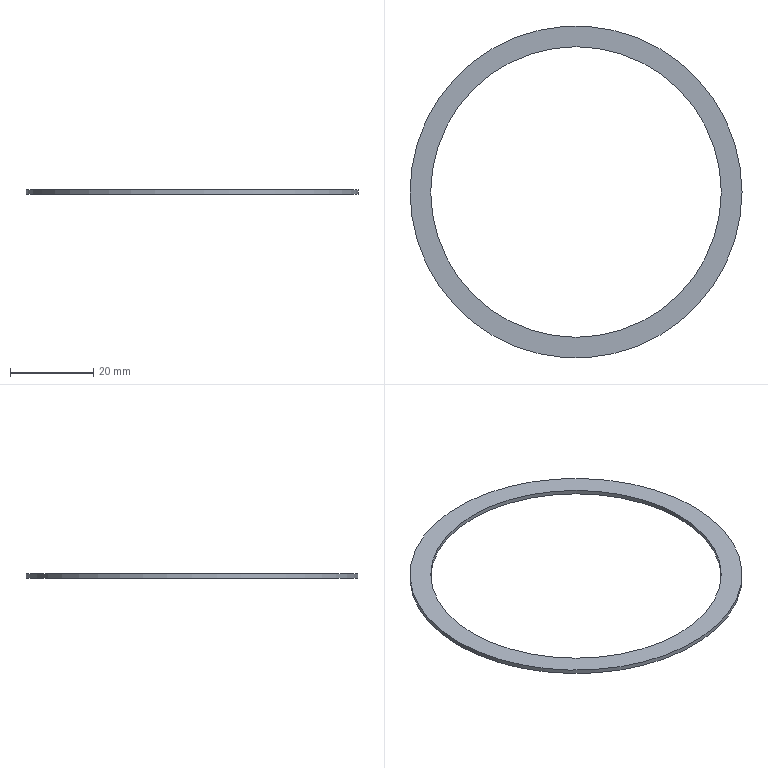Component | NX | BONNET_GASKET | 1 solid | 4 faces | box 80 x 80 x 1 mm | volume 1178 mm3 | plane 2 | cylinder 2 | commonest cylinder face diameters 80 x1 70 x1
STEP:
#1=CARTESIAN_POINT('',(0.,0.,0.));
#2=DIRECTION('',(0.,0.,1.));
#3=DIRECTION('',(1.,0.,0.));
#4=AXIS2_PLACEMENT_3D('',#1,#2,#3);
#5=CARTESIAN_POINT('',(35.,0.,-3.));
#6=VERTEX_POINT('',#5);
#7=CARTESIAN_POINT('',(0.,0.,-3.));
#8=DIRECTION('',(0.,0.,-1.));
#9=DIRECTION('',(1.,0.,0.));
#10=AXIS2_PLACEMENT_3D('',#7,#8,#9);
#11=CIRCLE('',#10,35.);
#12=CARTESIAN_POINT('',(0.,0.,-3.));
#13=DIRECTION('',(0.,0.,1.));
#14=DIRECTION('',(1.,0.,0.));
#15=AXIS2_PLACEMENT_3D('',#12,#13,#14);
#16=PLANE('',#15);
#17=CARTESIAN_POINT('',(35.,0.));
#18=CARTESIAN_POINT('',(35.,-60.622));
#19=CARTESIAN_POINT('',(-17.5,-30.311));
#20=CARTESIAN_POINT('',(-70.,-0.));
#21=CARTESIAN_POINT('',(-17.5,30.311));
#22=CARTESIAN_POINT('',(35.,60.622));
#23=CARTESIAN_POINT('',(35.,0.));
#24=(BOUNDED_CURVE()B_SPLINE_CURVE(2,(#17,#18,#19,#20,#21,#22,#23),.UNSPECIFIED.,.T.,.F.)B_SPLINE_CURVE_WITH_KNOTS((1,2,2,2,2,1),(-2.094,0.,2.094,4.189,6.283,8.378),.UNSPECIFIED.)CURVE()GEOMETRIC_REPRESENTATION_ITEM()RATIONAL_B_SPLINE_CURVE((1.,0.5,1.,0.5,1.,0.5,1.))REPRESENTATION_ITEM(''));
#25=(GEOMETRIC_REPRESENTATION_CONTEXT(2)PARAMETRIC_REPRESENTATION_CONTEXT()REPRESENTATION_CONTEXT('',''));
#26=DEFINITIONAL_REPRESENTATION('',(#24),#25);
#27=PCURVE('',#16,#26);
#28=CARTESIAN_POINT('',(0.,0.,-3.));
#29=DIRECTION('',(0.,0.,-1.));
#30=DIRECTION('',(1.,0.,0.));
#31=AXIS2_PLACEMENT_3D('',#28,#29,#30);
#32=CYLINDRICAL_SURFACE('',#31,35.);
#33=CARTESIAN_POINT('',(0.,0.));
#34=DIRECTION('',(1.,0.));
#35=VECTOR('',#34,1.);
#36=LINE('',#33,#35);
#37=(GEOMETRIC_REPRESENTATION_CONTEXT(2)PARAMETRIC_REPRESENTATION_CONTEXT()REPRESENTATION_CONTEXT('',''));
#38=DEFINITIONAL_REPRESENTATION('',(#36),#37);
#39=PCURVE('',#32,#38);
#40=SURFACE_CURVE('',#11,(#27,#39),.PCURVE_S1.);
#41=EDGE_CURVE('',#6,#6,#40,.T.);
#42=ORIENTED_EDGE('',*,*,#41,.T.);
#43=EDGE_LOOP('',(#42));
#44=FACE_BOUND('',#43,.T.);
#45=CARTESIAN_POINT('',(40.,0.,-3.));
#46=VERTEX_POINT('',#45);
#47=CARTESIAN_POINT('',(0.,0.,-3.));
#48=DIRECTION('',(0.,0.,-1.));
#49=DIRECTION('',(1.,0.,0.));
#50=AXIS2_PLACEMENT_3D('',#47,#48,#49);
#51=CIRCLE('',#50,40.);
#52=CARTESIAN_POINT('',(40.,0.));
#53=CARTESIAN_POINT('',(40.,-69.282));
#54=CARTESIAN_POINT('',(-20.,-34.641));
#55=CARTESIAN_POINT('',(-80.,-0.));
#56=CARTESIAN_POINT('',(-20.,34.641));
#57=CARTESIAN_POINT('',(40.,69.282));
#58=CARTESIAN_POINT('',(40.,0.));
#59=(BOUNDED_CURVE()B_SPLINE_CURVE(2,(#52,#53,#54,#55,#56,#57,#58),.UNSPECIFIED.,.T.,.F.)B_SPLINE_CURVE_WITH_KNOTS((1,2,2,2,2,1),(-2.094,0.,2.094,4.189,6.283,8.378),.UNSPECIFIED.)CURVE()GEOMETRIC_REPRESENTATION_ITEM()RATIONAL_B_SPLINE_CURVE((1.,0.5,1.,0.5,1.,0.5,1.))REPRESENTATION_ITEM(''));
#60=(GEOMETRIC_REPRESENTATION_CONTEXT(2)PARAMETRIC_REPRESENTATION_CONTEXT()REPRESENTATION_CONTEXT('',''));
#61=DEFINITIONAL_REPRESENTATION('',(#59),#60);
#62=PCURVE('',#16,#61);
#63=CARTESIAN_POINT('',(0.,0.,-4.));
#64=DIRECTION('',(0.,0.,1.));
#65=DIRECTION('',(1.,0.,0.));
#66=AXIS2_PLACEMENT_3D('',#63,#64,#65);
#67=CYLINDRICAL_SURFACE('',#66,40.);
#68=CARTESIAN_POINT('',(6.283,1.));
#69=DIRECTION('',(-1.,0.));
#70=VECTOR('',#69,1.);
#71=LINE('',#68,#70);
#72=(GEOMETRIC_REPRESENTATION_CONTEXT(2)PARAMETRIC_REPRESENTATION_CONTEXT()REPRESENTATION_CONTEXT('',''));
#73=DEFINITIONAL_REPRESENTATION('',(#71),#72);
#74=PCURVE('',#67,#73);
#75=SURFACE_CURVE('',#51,(#62,#74),.PCURVE_S1.);
#76=EDGE_CURVE('',#46,#46,#75,.T.);
#77=ORIENTED_EDGE('',*,*,#76,.F.);
#78=EDGE_LOOP('',(#77));
#79=FACE_BOUND('',#78,.T.);
#80=ADVANCED_FACE('',(#44,#79),#16,.T.);
#81=CARTESIAN_POINT('',(35.,0.,-4.));
#82=VERTEX_POINT('',#81);
#83=CARTESIAN_POINT('',(0.,0.,-4.));
#84=DIRECTION('',(0.,0.,1.));
#85=DIRECTION('',(1.,0.,0.));
#86=AXIS2_PLACEMENT_3D('',#83,#84,#85);
#87=CIRCLE('',#86,35.);
#88=CARTESIAN_POINT('',(0.,0.,-4.));
#89=DIRECTION('',(0.,0.,-1.));
#90=DIRECTION('',(-1.,0.,0.));
#91=AXIS2_PLACEMENT_3D('',#88,#89,#90);
#92=PLANE('',#91);
#93=CARTESIAN_POINT('',(-35.,0.));
#94=CARTESIAN_POINT('',(-35.,60.622));
#95=CARTESIAN_POINT('',(17.5,30.311));
#96=CARTESIAN_POINT('',(70.,0.));
#97=CARTESIAN_POINT('',(17.5,-30.311));
#98=CARTESIAN_POINT('',(-35.,-60.622));
#99=CARTESIAN_POINT('',(-35.,0.));
#100=(BOUNDED_CURVE()B_SPLINE_CURVE(2,(#93,#94,#95,#96,#97,#98,#99),.UNSPECIFIED.,.T.,.F.)B_SPLINE_CURVE_WITH_KNOTS((1,2,2,2,2,1),(-2.094,0.,2.094,4.189,6.283,8.378),.UNSPECIFIED.)CURVE()GEOMETRIC_REPRESENTATION_ITEM()RATIONAL_B_SPLINE_CURVE((1.,0.5,1.,0.5,1.,0.5,1.))REPRESENTATION_ITEM(''));
#101=(GEOMETRIC_REPRESENTATION_CONTEXT(2)PARAMETRIC_REPRESENTATION_CONTEXT()REPRESENTATION_CONTEXT('',''));
#102=DEFINITIONAL_REPRESENTATION('',(#100),#101);
#103=PCURVE('',#92,#102);
#104=CARTESIAN_POINT('',(6.283,1.));
#105=DIRECTION('',(-1.,0.));
#106=VECTOR('',#105,1.);
#107=LINE('',#104,#106);
#108=(GEOMETRIC_REPRESENTATION_CONTEXT(2)PARAMETRIC_REPRESENTATION_CONTEXT()REPRESENTATION_CONTEXT('',''));
#109=DEFINITIONAL_REPRESENTATION('',(#107),#108);
#110=PCURVE('',#32,#109);
#111=SURFACE_CURVE('',#87,(#103,#110),.PCURVE_S1.);
#112=EDGE_CURVE('',#82,#82,#111,.T.);
#113=ORIENTED_EDGE('',*,*,#112,.T.);
#114=EDGE_LOOP('',(#113));
#115=FACE_BOUND('',#114,.T.);
#116=CARTESIAN_POINT('',(40.,0.,-4.));
#117=VERTEX_POINT('',#116);
#118=CARTESIAN_POINT('',(0.,0.,-4.));
#119=DIRECTION('',(0.,0.,1.));
#120=DIRECTION('',(1.,0.,0.));
#121=AXIS2_PLACEMENT_3D('',#118,#119,#120);
#122=CIRCLE('',#121,40.);
#123=CARTESIAN_POINT('',(-40.,0.));
#124=CARTESIAN_POINT('',(-40.,69.282));
#125=CARTESIAN_POINT('',(20.,34.641));
#126=CARTESIAN_POINT('',(80.,0.));
#127=CARTESIAN_POINT('',(20.,-34.641));
#128=CARTESIAN_POINT('',(-40.,-69.282));
#129=CARTESIAN_POINT('',(-40.,0.));
#130=(BOUNDED_CURVE()B_SPLINE_CURVE(2,(#123,#124,#125,#126,#127,#128,#129),.UNSPECIFIED.,.T.,.F.)B_SPLINE_CURVE_WITH_KNOTS((1,2,2,2,2,1),(-2.094,0.,2.094,4.189,6.283,8.378),.UNSPECIFIED.)CURVE()GEOMETRIC_REPRESENTATION_ITEM()RATIONAL_B_SPLINE_CURVE((1.,0.5,1.,0.5,1.,0.5,1.))REPRESENTATION_ITEM(''));
#131=(GEOMETRIC_REPRESENTATION_CONTEXT(2)PARAMETRIC_REPRESENTATION_CONTEXT()REPRESENTATION_CONTEXT('',''));
#132=DEFINITIONAL_REPRESENTATION('',(#130),#131);
#133=PCURVE('',#92,#132);
#134=CARTESIAN_POINT('',(0.,0.));
#135=DIRECTION('',(1.,0.));
#136=VECTOR('',#135,1.);
#137=LINE('',#134,#136);
#138=(GEOMETRIC_REPRESENTATION_CONTEXT(2)PARAMETRIC_REPRESENTATION_CONTEXT()REPRESENTATION_CONTEXT('',''));
#139=DEFINITIONAL_REPRESENTATION('',(#137),#138);
#140=PCURVE('',#67,#139);
#141=SURFACE_CURVE('',#122,(#133,#140),.PCURVE_S1.);
#142=EDGE_CURVE('',#117,#117,#141,.T.);
#143=ORIENTED_EDGE('',*,*,#142,.F.);
#144=EDGE_LOOP('',(#143));
#145=FACE_BOUND('',#144,.T.);
#146=ADVANCED_FACE('',(#115,#145),#92,.T.);
#147=ORIENTED_EDGE('',*,*,#76,.T.);
#148=CARTESIAN_POINT('',(40.,-0.,-4.));
#149=CARTESIAN_POINT('',(40.,-0.,-3.));
#150=B_SPLINE_CURVE_WITH_KNOTS('',1,(#148,#149),.UNSPECIFIED.,.F.,.F.,(2,2),(0.,1.),.PIECEWISE_BEZIER_KNOTS.);
#151=CARTESIAN_POINT('',(0.,0.));
#152=DIRECTION('',(0.,1.));
#153=VECTOR('',#152,1.);
#154=LINE('',#151,#153);
#155=(GEOMETRIC_REPRESENTATION_CONTEXT(2)PARAMETRIC_REPRESENTATION_CONTEXT()REPRESENTATION_CONTEXT('',''));
#156=DEFINITIONAL_REPRESENTATION('',(#154),#155);
#157=PCURVE('',#67,#156);
#158=CARTESIAN_POINT('',(6.283,0.));
#159=DIRECTION('',(0.,1.));
#160=VECTOR('',#159,1.);
#161=LINE('',#158,#160);
#162=(GEOMETRIC_REPRESENTATION_CONTEXT(2)PARAMETRIC_REPRESENTATION_CONTEXT()REPRESENTATION_CONTEXT('',''));
#163=DEFINITIONAL_REPRESENTATION('',(#161),#162);
#164=PCURVE('',#67,#163);
#165=SEAM_CURVE('',#150,(#157,#164),.PCURVE_S1.);
#166=EDGE_CURVE('',#117,#46,#165,.T.);
#167=ORIENTED_EDGE('',*,*,#166,.F.);
#168=ORIENTED_EDGE('',*,*,#142,.T.);
#169=ORIENTED_EDGE('',*,*,#166,.T.);
#170=EDGE_LOOP('',(#147,#167,#168,#169));
#171=FACE_BOUND('',#170,.T.);
#172=ADVANCED_FACE('',(#171),#67,.T.);
#173=ORIENTED_EDGE('',*,*,#112,.T.);
#174=CARTESIAN_POINT('',(35.,0.,-3.));
#175=CARTESIAN_POINT('',(35.,0.,-4.));
#176=B_SPLINE_CURVE_WITH_KNOTS('',1,(#174,#175),.UNSPECIFIED.,.F.,.F.,(2,2),(0.,1.),.PIECEWISE_BEZIER_KNOTS.);
#177=CARTESIAN_POINT('',(0.,0.));
#178=DIRECTION('',(0.,1.));
#179=VECTOR('',#178,1.);
#180=LINE('',#177,#179);
#181=(GEOMETRIC_REPRESENTATION_CONTEXT(2)PARAMETRIC_REPRESENTATION_CONTEXT()REPRESENTATION_CONTEXT('',''));
#182=DEFINITIONAL_REPRESENTATION('',(#180),#181);
#183=PCURVE('',#32,#182);
#184=CARTESIAN_POINT('',(6.283,0.));
#185=DIRECTION('',(0.,1.));
#186=VECTOR('',#185,1.);
#187=LINE('',#184,#186);
#188=(GEOMETRIC_REPRESENTATION_CONTEXT(2)PARAMETRIC_REPRESENTATION_CONTEXT()REPRESENTATION_CONTEXT('',''));
#189=DEFINITIONAL_REPRESENTATION('',(#187),#188);
#190=PCURVE('',#32,#189);
#191=SEAM_CURVE('',#176,(#183,#190),.PCURVE_S1.);
#192=EDGE_CURVE('',#6,#82,#191,.T.);
#193=ORIENTED_EDGE('',*,*,#192,.F.);
#194=ORIENTED_EDGE('',*,*,#41,.T.);
#195=ORIENTED_EDGE('',*,*,#192,.T.);
#196=EDGE_LOOP('',(#173,#193,#194,#195));
#197=FACE_BOUND('',#196,.F.);
#198=ADVANCED_FACE('',(#197),#32,.F.);
#199=CLOSED_SHELL('',(#80,#146,#172,#198));
#200=MANIFOLD_SOLID_BREP('',#199);
#201=(LENGTH_UNIT()NAMED_UNIT(*)SI_UNIT(.MILLI.,.METRE.));
#202=UNCERTAINTY_MEASURE_WITH_UNIT(LENGTH_MEASURE(0.00001),#201,'','');
#203=(NAMED_UNIT(*)PLANE_ANGLE_UNIT()SI_UNIT($,.RADIAN.));
#204=(NAMED_UNIT(*)SI_UNIT($,.STERADIAN.)SOLID_ANGLE_UNIT());
#205=(GEOMETRIC_REPRESENTATION_CONTEXT(3)GLOBAL_UNCERTAINTY_ASSIGNED_CONTEXT((#202))GLOBAL_UNIT_ASSIGNED_CONTEXT((#201,#203,#204))REPRESENTATION_CONTEXT('',''));
#206=ADVANCED_BREP_SHAPE_REPRESENTATION('',(#4,#200),#205);